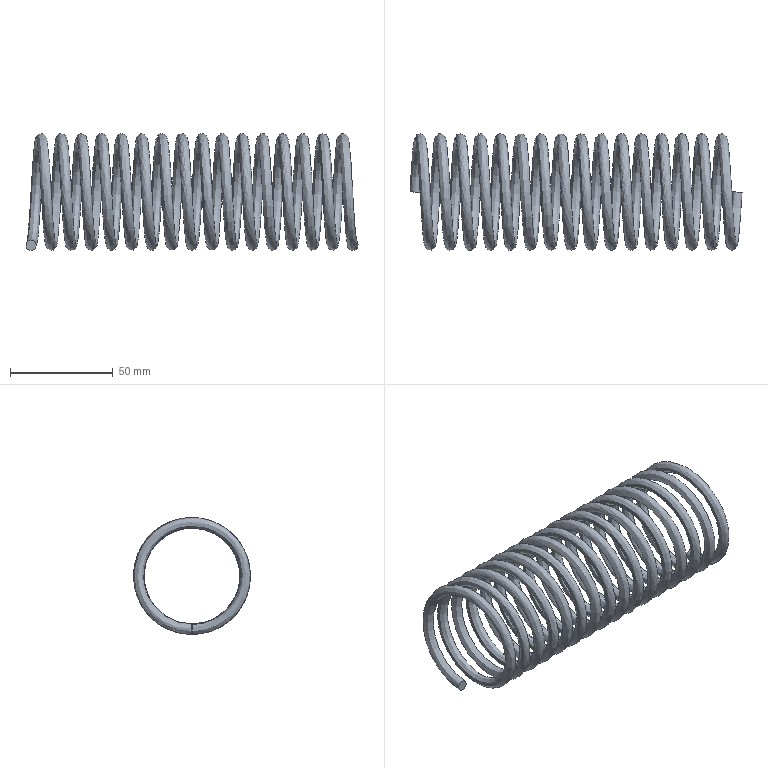Component | NX | SPRING | 1 solid | 3 faces | volume 51282 mm3 | plane 2 | spline 1